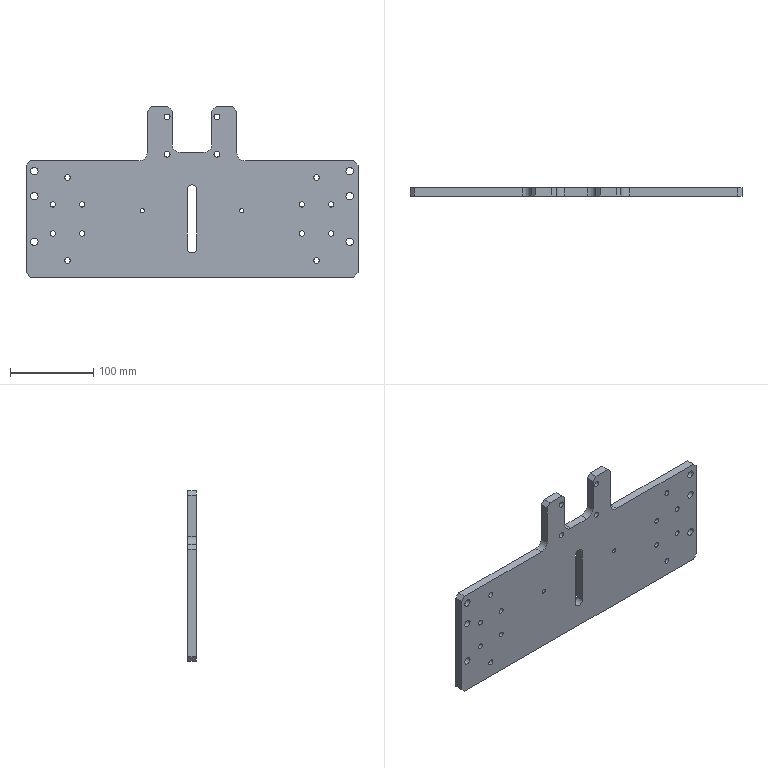Component | SolidWorks | OT-0100-004(BasePlate)-1 | 1 solid | 78 faces | box 400 x 10 x 205 mm | volume 584271 mm3 | cylinder 54 | plane 24 | commonest cylinder face diameters 6.5 x16 9 x12 6.8 x8 7 x8 5 x4 20 x4 12 x2
build123d program:
from build123d import *

# Parameters (mm, degrees)
SKETCH1_R             = 4.5
BOSS_EXTRUDE1_DEPTH   = 10
CUT_EXTRUDE1_REACH    = 288.575
SKETCH2_R             = 3.5
M8_TAPPED_HOLE1_D     = 6.8
M8_TAPPED_HOLE1_DEPTH = 19.75
M8_TAPPED_HOLE1_TIP   = 2.043
CHAMFER1_SIZE         = 5
CUT_EXTRUDE2_REACH    = 288.575
SKETCH10_R            = 3.25
CUT_EXTRUDE3_REACH    = 288.575
SKETCH11_R            = 4.5
M6_TAPPED_HOLE1_D     = 5
M6_TAPPED_HOLE1_DEPTH = 15
M6_TAPPED_HOLE1_TIP   = 1.502


with BuildPart() as part:
    # Sketch1 → Boss-Extrude1 (new body)
    with BuildSketch(Plane(origin=(0, 0, 0), x_dir=(1, 0, 0), z_dir=(0, 1, 0))):
        with BuildLine():
            Line((0, 200), (0, -200))
            Line((0, -200), (140, -200))
            Line((140, -200), (140, -64))
            ThreePointArc((140, -64), (142.929, -56.929), (150, -54))
            Line((150, -54), (205, -54))
            Line((205, -54), (205, -24))
            Line((205, -24), (160, -24))
            ThreePointArc((160, -24), (152.929, -21.071), (150, -14))
            Line((150, -14), (150, 14))
            ThreePointArc((150, 14), (152.929, 21.071), (160, 24))
            Line((160, 24), (205, 24))
            Line((205, 24), (205, 54))
            Line((205, 54), (150, 54))
            ThreePointArc((150, 54), (142.929, 56.929), (140, 64))
            Line((140, 64), (140, 200))
            Line((140, 200), (0, 200))
        make_face()
        with Locations(Location((42.5, 190, 0), (0, 0, 270))):
            Circle(SKETCH1_R, mode=Mode.SUBTRACT)
        with Locations(Location((97.5, 190, 0), (0, 0, 270))):
            Circle(SKETCH1_R, mode=Mode.SUBTRACT)
        with Locations(Location((97.5, -190, 0), (0, 0, 90))):
            Circle(SKETCH1_R, mode=Mode.SUBTRACT)
        with Locations(Location((42.5, -190, 0), (0, 0, 90))):
            Circle(SKETCH1_R, mode=Mode.SUBTRACT)
        with BuildLine():
            Line((35, 6), (105, 6))
            ThreePointArc((105, 6), (111, 0), (105, -6))
            Line((105, -6), (35, -6))
            ThreePointArc((35, -6), (29, 0), (35, 6))
        make_face(mode=Mode.SUBTRACT)
    extrude(amount=BOSS_EXTRUDE1_DEPTH)

    # Sketch2 → Cut-Extrude1 (cut, up to next)
    with BuildSketch(Plane(origin=(0, 10, 0), x_dir=(1, 0, 0), z_dir=(0, 1, 0)), mode=Mode.PRIVATE) as cut_extrude1_sk1:
        with Locations(Location((148, 30, 0), (0, 0, 270))):
            Circle(SKETCH2_R)
    cut_extrude1_tool1 = extrude(cut_extrude1_sk1.sketch, amount=-CUT_EXTRUDE1_REACH, mode=Mode.PRIVATE) & part.part
    # Sketch2 → Cut-Extrude1 (cut, up to next)
    with BuildSketch(Plane(origin=(0, 10, 0), x_dir=(1, 0, 0), z_dir=(0, 1, 0)), mode=Mode.PRIVATE) as cut_extrude1_sk2:
        with Locations(Location((193, 30, 0), (0, 0, 270))):
            Circle(SKETCH2_R)
    cut_extrude1_tool2 = extrude(cut_extrude1_sk2.sketch, amount=-CUT_EXTRUDE1_REACH, mode=Mode.PRIVATE) & part.part
    # Sketch2 → Cut-Extrude1 (cut, up to next)
    with BuildSketch(Plane(origin=(0, 10, 0), x_dir=(1, 0, 0), z_dir=(0, 1, 0)), mode=Mode.PRIVATE) as cut_extrude1_sk3:
        with Locations(Location((193, -30, 0), (0, 0, 90))):
            Circle(SKETCH2_R)
    cut_extrude1_tool3 = extrude(cut_extrude1_sk3.sketch, amount=-CUT_EXTRUDE1_REACH, mode=Mode.PRIVATE) & part.part
    # Sketch2 → Cut-Extrude1 (cut, up to next)
    with BuildSketch(Plane(origin=(0, 10, 0), x_dir=(1, 0, 0), z_dir=(0, 1, 0)), mode=Mode.PRIVATE) as cut_extrude1_sk4:
        with Locations(Location((148, -30, 0), (0, 0, 90))):
            Circle(SKETCH2_R)
    cut_extrude1_tool4 = extrude(cut_extrude1_sk4.sketch, amount=-CUT_EXTRUDE1_REACH, mode=Mode.PRIVATE) & part.part
    add(cut_extrude1_tool1.solids().sort_by_distance((148, 10, -30))[0], mode=Mode.SUBTRACT)
    add(cut_extrude1_tool2.solids().sort_by_distance((193, 10, -30))[0], mode=Mode.SUBTRACT)
    add(cut_extrude1_tool3.solids().sort_by_distance((193, 10, 30))[0], mode=Mode.SUBTRACT)
    add(cut_extrude1_tool4.solids().sort_by_distance((148, 10, 30))[0], mode=Mode.SUBTRACT)

    # M8 Tapped Hole1
    with Locations(Plane(origin=(0, 10, 0), x_dir=(1, 0, 0), z_dir=(0, 1, 0))):
        with Locations((20, -150), (120, -150), (120, 150), (20, 150)):
            Hole(M8_TAPPED_HOLE1_D / 2, depth=M8_TAPPED_HOLE1_DEPTH)
            with Locations((0, 0, -(M8_TAPPED_HOLE1_DEPTH + M8_TAPPED_HOLE1_TIP / 2))):  # 118° drill point
                Cone(0, M8_TAPPED_HOLE1_D / 2, M8_TAPPED_HOLE1_TIP, mode=Mode.SUBTRACT)

    # Chamfer1
    chamfer1_edges = [part.edges().sort_by_distance(p)[0] for p in [
        (0, 5, 200),
        (0, 5, -200),
        (140, 5, -200),
        (205, 5, -54),
        (205, 5, -24),
        (205, 5, 24),
        (205, 5, 54),
        (140, 5, 200),
    ]]
    chamfer(chamfer1_edges, length=CHAMFER1_SIZE)

    # Sketch10 → Cut-Extrude2 (cut, up to next)
    with BuildSketch(Plane(origin=(0, 10, 0), x_dir=(1, 0, 0), z_dir=(0, 1, 0)), mode=Mode.PRIVATE) as cut_extrude2_sk1:
        with Locations(Location((52.5, -132.5, 0), (0, 0, 270))):
            Circle(SKETCH10_R)
    cut_extrude2_tool1 = extrude(cut_extrude2_sk1.sketch, amount=-CUT_EXTRUDE2_REACH, mode=Mode.PRIVATE) & part.part
    # Sketch10 → Cut-Extrude2 (cut, up to next)
    with BuildSketch(Plane(origin=(0, 10, 0), x_dir=(1, 0, 0), z_dir=(0, 1, 0)), mode=Mode.PRIVATE) as cut_extrude2_sk2:
        with Locations(Location((52.5, -167.5, 0), (0, 0, 270))):
            Circle(SKETCH10_R)
    cut_extrude2_tool2 = extrude(cut_extrude2_sk2.sketch, amount=-CUT_EXTRUDE2_REACH, mode=Mode.PRIVATE) & part.part
    # Sketch10 → Cut-Extrude2 (cut, up to next)
    with BuildSketch(Plane(origin=(0, 10, 0), x_dir=(1, 0, 0), z_dir=(0, 1, 0)), mode=Mode.PRIVATE) as cut_extrude2_sk3:
        with Locations(Location((87.5, -167.5, 0), (0, 0, 90))):
            Circle(SKETCH10_R)
    cut_extrude2_tool3 = extrude(cut_extrude2_sk3.sketch, amount=-CUT_EXTRUDE2_REACH, mode=Mode.PRIVATE) & part.part
    # Sketch10 → Cut-Extrude2 (cut, up to next)
    with BuildSketch(Plane(origin=(0, 10, 0), x_dir=(1, 0, 0), z_dir=(0, 1, 0)), mode=Mode.PRIVATE) as cut_extrude2_sk4:
        with Locations(Location((87.5, -132.5, 0), (0, 0, 90))):
            Circle(SKETCH10_R)
    cut_extrude2_tool4 = extrude(cut_extrude2_sk4.sketch, amount=-CUT_EXTRUDE2_REACH, mode=Mode.PRIVATE) & part.part
    # Sketch10 → Cut-Extrude2 (cut, up to next)
    with BuildSketch(Plane(origin=(0, 10, 0), x_dir=(1, 0, 0), z_dir=(0, 1, 0)), mode=Mode.PRIVATE) as cut_extrude2_sk5:
        with Locations(Location((87.5, 132.5, 0), (0, 0, 270))):
            Circle(SKETCH10_R)
    cut_extrude2_tool5 = extrude(cut_extrude2_sk5.sketch, amount=-CUT_EXTRUDE2_REACH, mode=Mode.PRIVATE) & part.part
    # Sketch10 → Cut-Extrude2 (cut, up to next)
    with BuildSketch(Plane(origin=(0, 10, 0), x_dir=(1, 0, 0), z_dir=(0, 1, 0)), mode=Mode.PRIVATE) as cut_extrude2_sk6:
        with Locations(Location((87.5, 167.5, 0), (0, 0, 270))):
            Circle(SKETCH10_R)
    cut_extrude2_tool6 = extrude(cut_extrude2_sk6.sketch, amount=-CUT_EXTRUDE2_REACH, mode=Mode.PRIVATE) & part.part
    # Sketch10 → Cut-Extrude2 (cut, up to next)
    with BuildSketch(Plane(origin=(0, 10, 0), x_dir=(1, 0, 0), z_dir=(0, 1, 0)), mode=Mode.PRIVATE) as cut_extrude2_sk7:
        with Locations(Location((52.5, 167.5, 0), (0, 0, 90))):
            Circle(SKETCH10_R)
    cut_extrude2_tool7 = extrude(cut_extrude2_sk7.sketch, amount=-CUT_EXTRUDE2_REACH, mode=Mode.PRIVATE) & part.part
    # Sketch10 → Cut-Extrude2 (cut, up to next)
    with BuildSketch(Plane(origin=(0, 10, 0), x_dir=(1, 0, 0), z_dir=(0, 1, 0)), mode=Mode.PRIVATE) as cut_extrude2_sk8:
        with Locations(Location((52.5, 132.5, 0), (0, 0, 90))):
            Circle(SKETCH10_R)
    cut_extrude2_tool8 = extrude(cut_extrude2_sk8.sketch, amount=-CUT_EXTRUDE2_REACH, mode=Mode.PRIVATE) & part.part
    add(cut_extrude2_tool1.solids().sort_by_distance((52.5, 10, 132.5))[0], mode=Mode.SUBTRACT)
    add(cut_extrude2_tool2.solids().sort_by_distance((52.5, 10, 167.5))[0], mode=Mode.SUBTRACT)
    add(cut_extrude2_tool3.solids().sort_by_distance((87.5, 10, 167.5))[0], mode=Mode.SUBTRACT)
    add(cut_extrude2_tool4.solids().sort_by_distance((87.5, 10, 132.5))[0], mode=Mode.SUBTRACT)
    add(cut_extrude2_tool5.solids().sort_by_distance((87.5, 10, -132.5))[0], mode=Mode.SUBTRACT)
    add(cut_extrude2_tool6.solids().sort_by_distance((87.5, 10, -167.5))[0], mode=Mode.SUBTRACT)
    add(cut_extrude2_tool7.solids().sort_by_distance((52.5, 10, -167.5))[0], mode=Mode.SUBTRACT)
    add(cut_extrude2_tool8.solids().sort_by_distance((52.5, 10, -132.5))[0], mode=Mode.SUBTRACT)

    # Sketch11 → Cut-Extrude3 (cut, up to next)
    with BuildSketch(Plane.XZ, mode=Mode.PRIVATE) as cut_extrude3_sk1:
        with Locations(Location((127.5, 190, 0), (0, 0, 270))):
            Circle(SKETCH11_R)
    cut_extrude3_tool1 = extrude(cut_extrude3_sk1.sketch, amount=-CUT_EXTRUDE3_REACH, mode=Mode.PRIVATE) & part.part
    # Sketch11 → Cut-Extrude3 (cut, up to next)
    with BuildSketch(Plane.XZ, mode=Mode.PRIVATE) as cut_extrude3_sk2:
        with Locations(Location((127.5, -190, 0), (0, 0, 270))):
            Circle(SKETCH11_R)
    cut_extrude3_tool2 = extrude(cut_extrude3_sk2.sketch, amount=-CUT_EXTRUDE3_REACH, mode=Mode.PRIVATE) & part.part
    add(cut_extrude3_tool1.solids().sort_by_distance((127.5, 0, 190))[0], mode=Mode.SUBTRACT)
    add(cut_extrude3_tool2.solids().sort_by_distance((127.5, 0, -190))[0], mode=Mode.SUBTRACT)

    # M6 Tapped Hole1
    with Locations(Plane(origin=(0, 10, 0), x_dir=(1, 0, 0), z_dir=(0, 1, 0))):
        with Locations((80, -60), (80, 60)):
            Hole(M6_TAPPED_HOLE1_D / 2, depth=M6_TAPPED_HOLE1_DEPTH)
            with Locations((0, 0, -(M6_TAPPED_HOLE1_DEPTH + M6_TAPPED_HOLE1_TIP / 2))):  # 118° drill point
                Cone(0, M6_TAPPED_HOLE1_D / 2, M6_TAPPED_HOLE1_TIP, mode=Mode.SUBTRACT)


solid = part.part

# Placed as in the assembly
solid = solid.moved(Location((200, 70, -70), (0, -90, 0)))